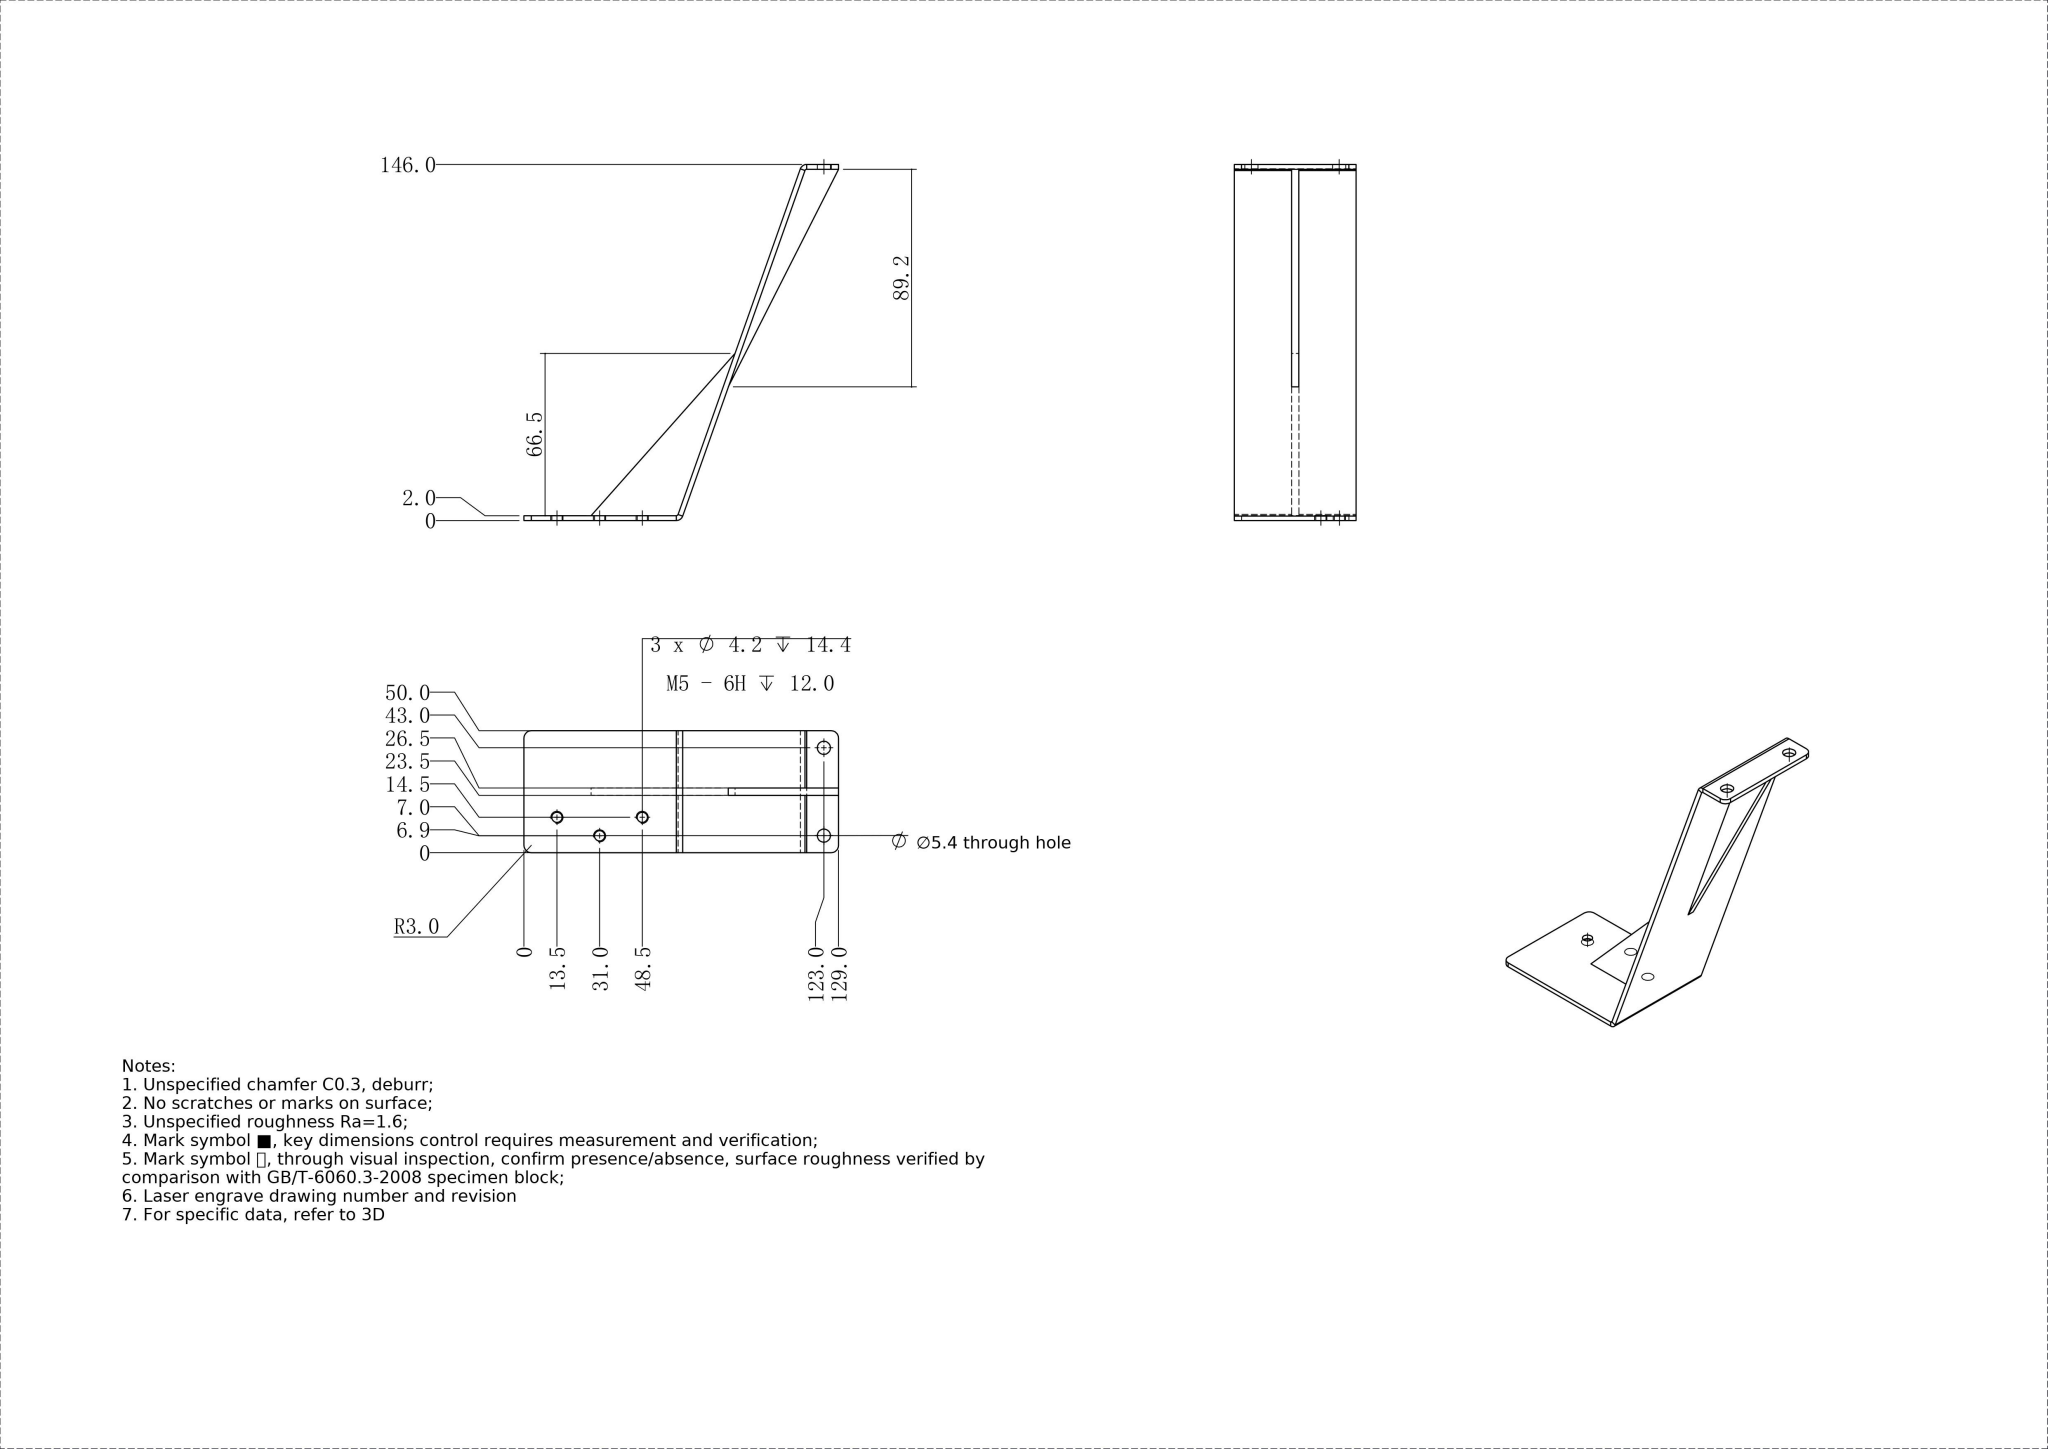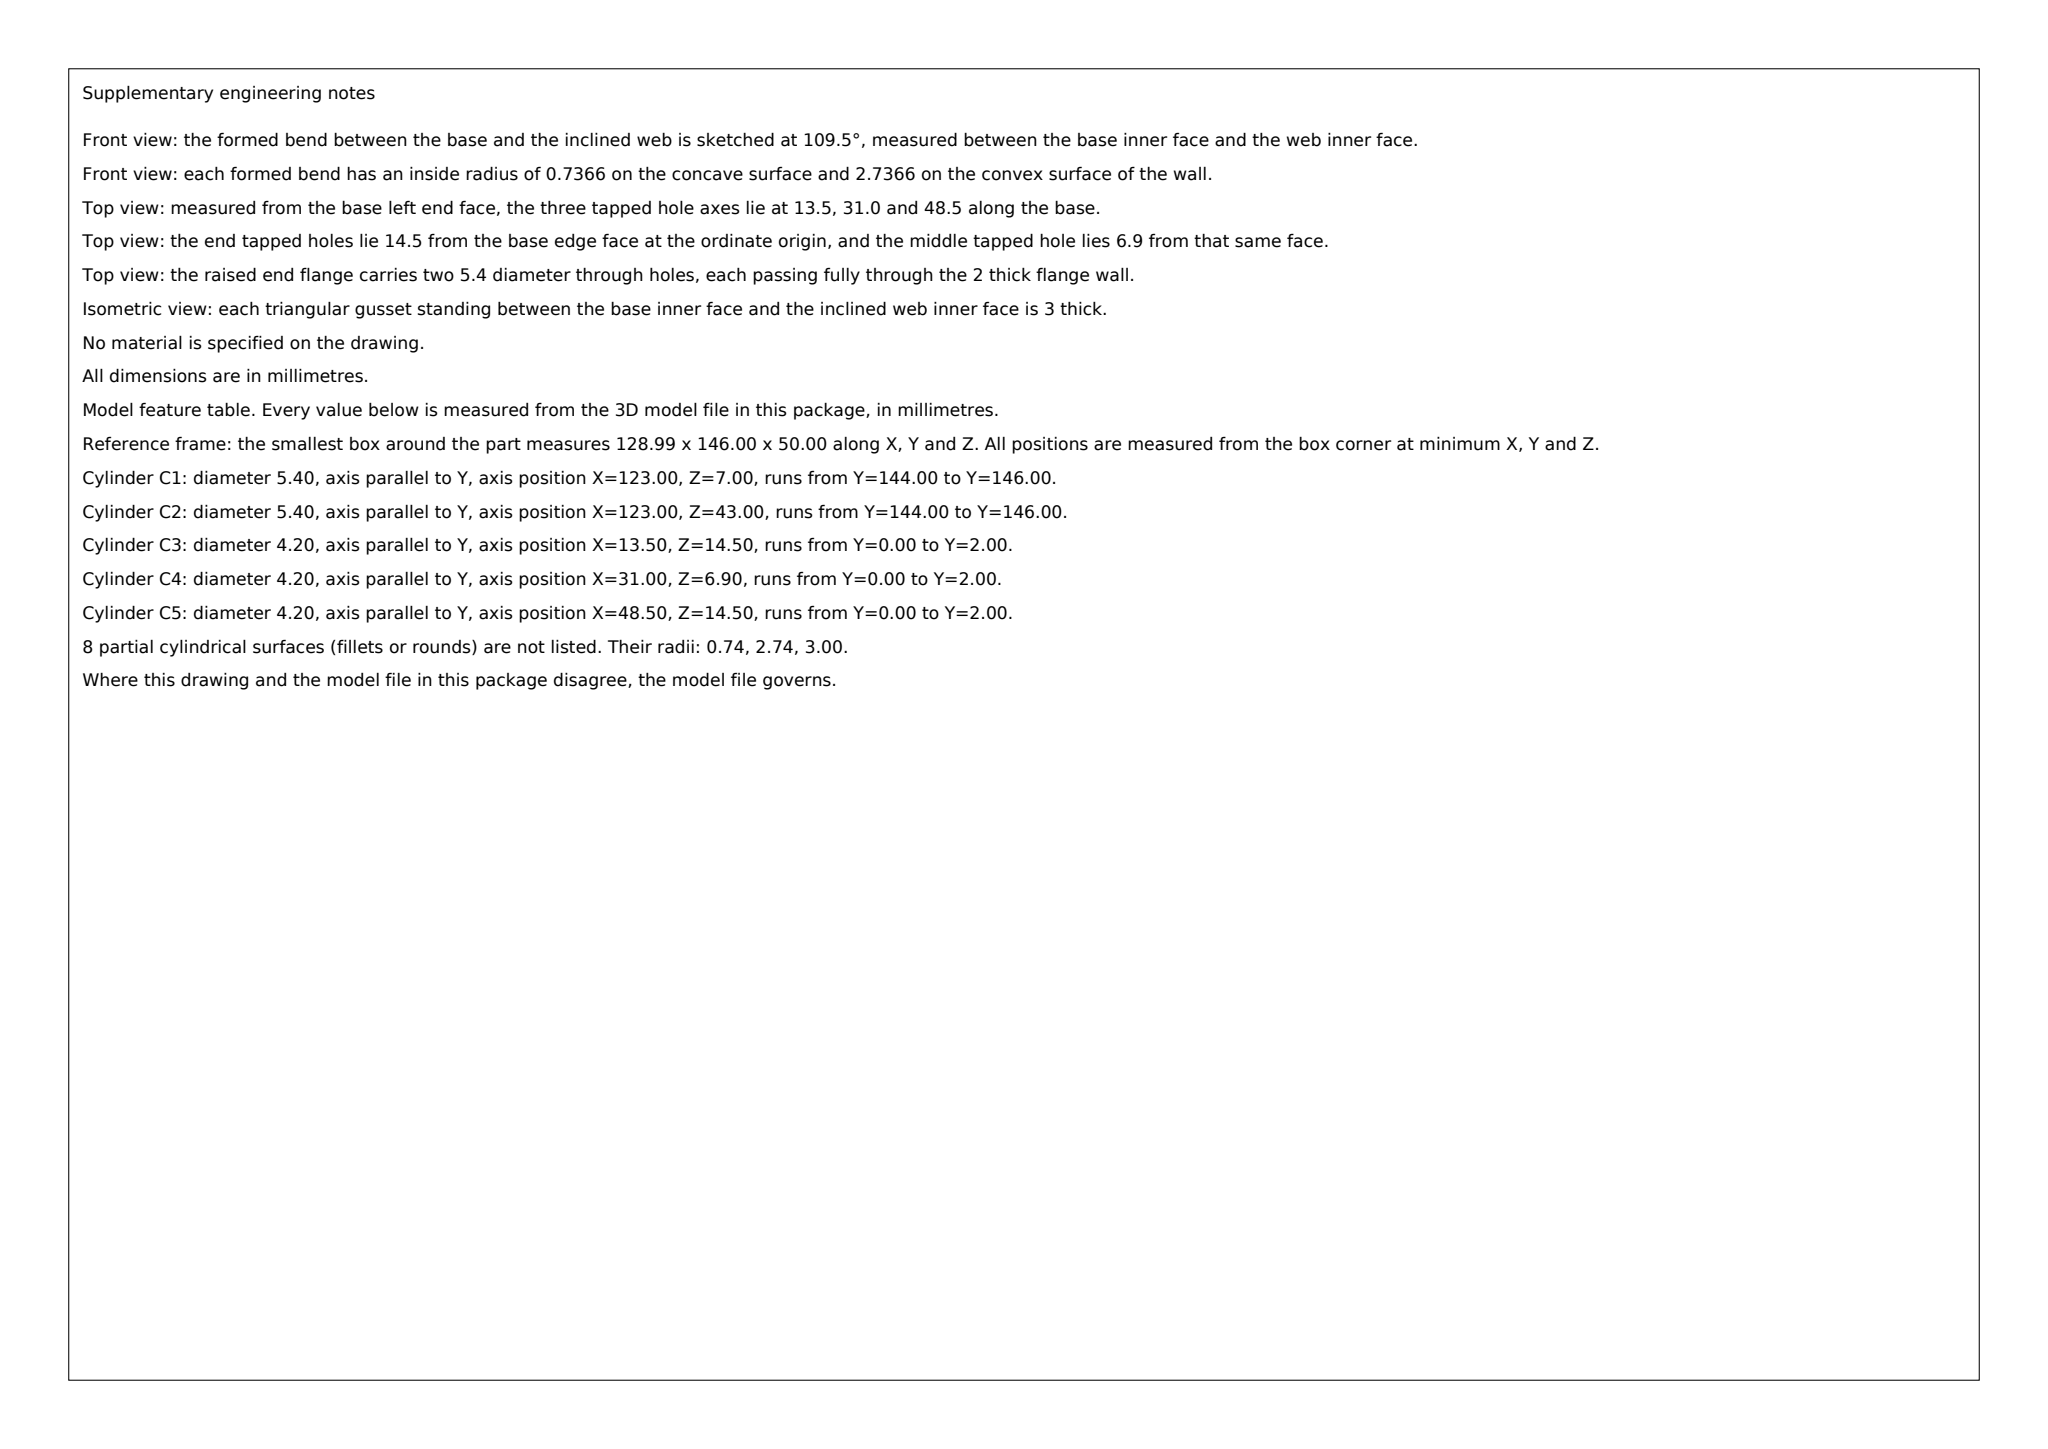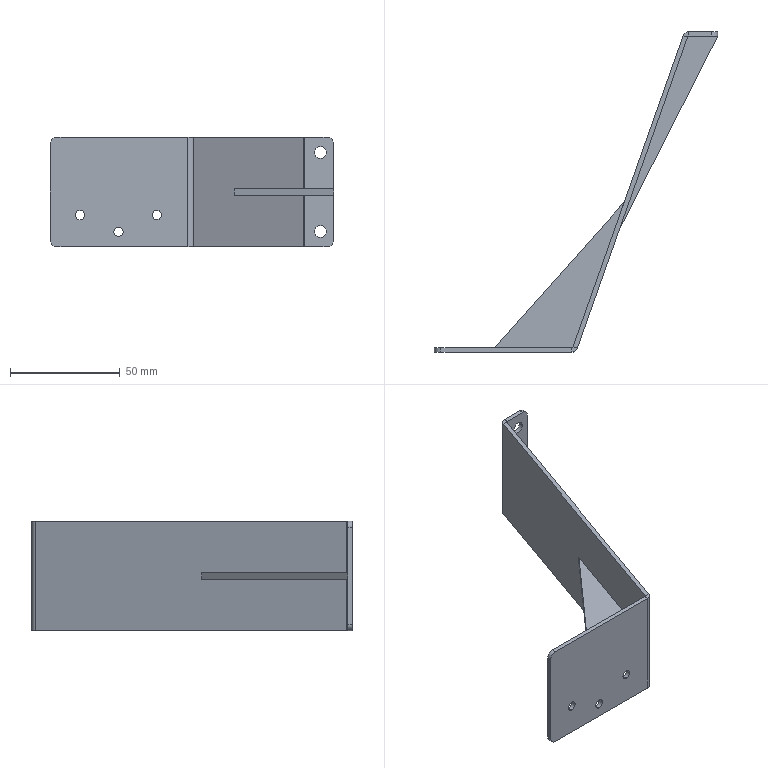Part | SolidWorks | mm | 1 solid | 45 faces | box 128.99 x 146 x 50 mm | volume 28182 mm3 | plane 25 | cylinder 20 | commonest cylinder face diameters 4.2 x6 5.4 x4 1.473 x4 6 x4 5.473 x2
Drawing notes:
4X R3.0 CORNERS: 2 AT BASE END, 2 AT TOP FLANGE | from the solid: Four Ø6.0 y-axis cyl len 2.0 at (3.0,3.0),(3.0,47.0),(125.99,3.0),(125.99,47.0) = R3.0
TOP FLANGE UNDER FACE 144.0 ABOVE BASE, FLANGE PAR TO BASE | from the solid: Y-normal planes y=0/2.0 (base) and y=144.0/146.0 (flange) parallel; bbox y=146.0
GUSSET RIB 3.0 THK, CTRD ON 50 WIDTH (Z 23.5-26.5), PROFILE PER FV | from the solid: axis_planes z=23.5 (2) and z=26.5 (2); bbox z=50; band 23.5-26.5 = 3.0 thk about z=25
SLOT 3.0 WIDE (Z 23.5-26.5) THRU INCL FACE, FULL LEN BTWN BENDS | from the solid: Same z=23.5/26.5 planes; bend fillet cyl Ø1.473 split 2 x 23.5 long at (62.48,2.74) and (115.93,143.26)